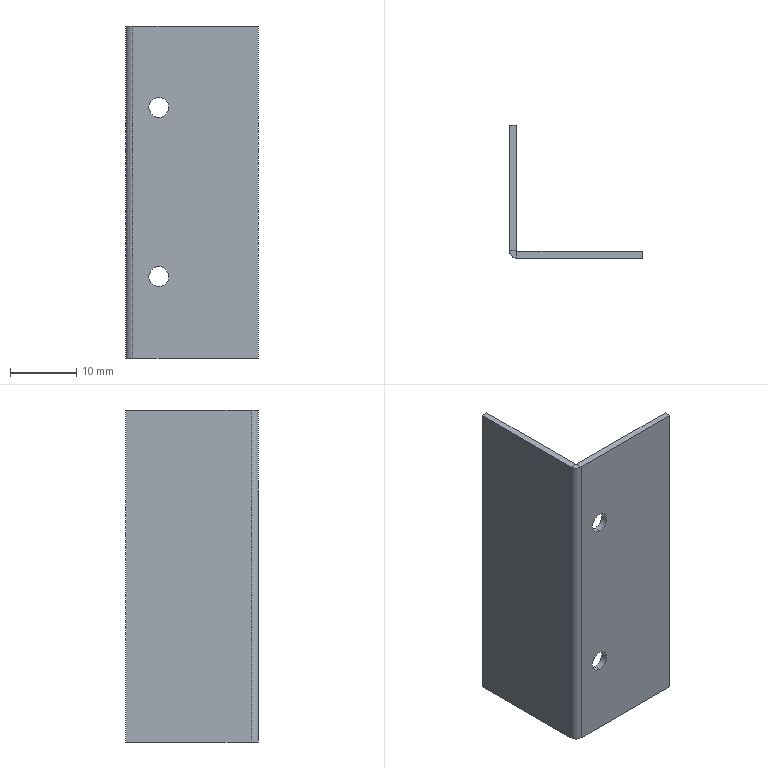Component | SolidWorks | CabinetWelding-1_LimitSwitchBracket-1 | 1 solid | 18 faces | box 20 x 20 x 50 mm | volume 1923 mm3 | plane 12 | cylinder 6 | commonest cylinder face diameters 3 x4 2.2 x1 0.2 x1
STEP:
#1=COLOUR_RGB('',0.7922,0.8196,0.9333);
#2=FILL_AREA_STYLE_COLOUR('',#1);
#3=FILL_AREA_STYLE('',(#2));
#4=SURFACE_STYLE_FILL_AREA(#3);
#5=SURFACE_SIDE_STYLE('',(#4));
#6=SURFACE_STYLE_USAGE(.BOTH.,#5);
#7=PRESENTATION_STYLE_ASSIGNMENT((#6));
#8=CARTESIAN_POINT('',(4.46,33.389,93.238));
#9=VERTEX_POINT('',#8);
#10=CARTESIAN_POINT('',(4.46,33.389,93.357));
#11=VERTEX_POINT('',#10);
#12=CARTESIAN_POINT('',(4.46,33.389,93.297));
#13=DIRECTION('',(-0.,1.,0.));
#14=DIRECTION('',(0.,0.,1.));
#15=AXIS2_PLACEMENT_3D('',#12,#13,#14);
#16=CIRCLE('',#15,0.05906);
#17=EDGE_CURVE('',#9,#11,#16,.T.);
#18=ORIENTED_EDGE('',*,*,#17,.F.);
#19=CARTESIAN_POINT('',(4.46,33.428,93.238));
#20=VERTEX_POINT('',#19);
#21=CARTESIAN_POINT('',(4.46,33.389,93.238));
#22=DIRECTION('',(-0.,1.,0.));
#23=VECTOR('',#22,39.37);
#24=LINE('',#21,#23);
#25=EDGE_CURVE('',#9,#20,#24,.T.);
#26=ORIENTED_EDGE('',*,*,#25,.T.);
#27=CARTESIAN_POINT('',(4.46,33.428,93.357));
#28=VERTEX_POINT('',#27);
#29=CARTESIAN_POINT('',(4.46,33.428,93.297));
#30=DIRECTION('',(-0.,1.,0.));
#31=DIRECTION('',(0.,0.,1.));
#32=AXIS2_PLACEMENT_3D('',#29,#30,#31);
#33=CIRCLE('',#32,0.05906);
#34=EDGE_CURVE('',#20,#28,#33,.T.);
#35=ORIENTED_EDGE('',*,*,#34,.T.);
#36=CARTESIAN_POINT('',(4.46,33.389,93.357));
#37=DIRECTION('',(-0.,1.,0.));
#38=VECTOR('',#37,39.37);
#39=LINE('',#36,#38);
#40=EDGE_CURVE('',#11,#28,#39,.T.);
#41=ORIENTED_EDGE('',*,*,#40,.F.);
#42=EDGE_LOOP('',(#18,#26,#35,#41));
#43=FACE_OUTER_BOUND('',#42,.T.);
#44=CARTESIAN_POINT('',(4.46,33.389,93.297));
#45=DIRECTION('',(-0.,1.,0.));
#46=DIRECTION('',(0.,0.,1.));
#47=AXIS2_PLACEMENT_3D('',#44,#45,#46);
#48=CYLINDRICAL_SURFACE('',#47,0.05906);
#49=ADVANCED_FACE('',(#43),#48,.F.);
#50=CARTESIAN_POINT('',(4.46,33.389,92.234));
#51=VERTEX_POINT('',#50);
#52=CARTESIAN_POINT('',(4.46,33.389,92.353));
#53=VERTEX_POINT('',#52);
#54=CARTESIAN_POINT('',(4.46,33.389,92.294));
#55=DIRECTION('',(-0.,1.,0.));
#56=DIRECTION('',(0.,0.,1.));
#57=AXIS2_PLACEMENT_3D('',#54,#55,#56);
#58=CIRCLE('',#57,0.05906);
#59=EDGE_CURVE('',#51,#53,#58,.T.);
#60=ORIENTED_EDGE('',*,*,#59,.F.);
#61=CARTESIAN_POINT('',(4.46,33.428,92.234));
#62=VERTEX_POINT('',#61);
#63=CARTESIAN_POINT('',(4.46,33.389,92.234));
#64=DIRECTION('',(-0.,1.,0.));
#65=VECTOR('',#64,39.37);
#66=LINE('',#63,#65);
#67=EDGE_CURVE('',#51,#62,#66,.T.);
#68=ORIENTED_EDGE('',*,*,#67,.T.);
#69=CARTESIAN_POINT('',(4.46,33.428,92.353));
#70=VERTEX_POINT('',#69);
#71=CARTESIAN_POINT('',(4.46,33.428,92.294));
#72=DIRECTION('',(-0.,1.,0.));
#73=DIRECTION('',(0.,0.,1.));
#74=AXIS2_PLACEMENT_3D('',#71,#72,#73);
#75=CIRCLE('',#74,0.05906);
#76=EDGE_CURVE('',#62,#70,#75,.T.);
#77=ORIENTED_EDGE('',*,*,#76,.T.);
#78=CARTESIAN_POINT('',(4.46,33.389,92.353));
#79=DIRECTION('',(-0.,1.,0.));
#80=VECTOR('',#79,39.37);
#81=LINE('',#78,#80);
#82=EDGE_CURVE('',#53,#70,#81,.T.);
#83=ORIENTED_EDGE('',*,*,#82,.F.);
#84=EDGE_LOOP('',(#60,#68,#77,#83));
#85=FACE_OUTER_BOUND('',#84,.T.);
#86=CARTESIAN_POINT('',(4.46,33.389,92.294));
#87=DIRECTION('',(-0.,1.,0.));
#88=DIRECTION('',(0.,0.,1.));
#89=AXIS2_PLACEMENT_3D('',#86,#87,#88);
#90=CYLINDRICAL_SURFACE('',#89,0.05906);
#91=ADVANCED_FACE('',(#85),#90,.F.);
#92=CARTESIAN_POINT('',(4.302,33.432,91.811));
#93=VERTEX_POINT('',#92);
#94=CARTESIAN_POINT('',(4.302,34.176,91.811));
#95=VERTEX_POINT('',#94);
#96=CARTESIAN_POINT('',(4.302,34.176,91.811));
#97=DIRECTION('',(-0.,1.,0.));
#98=VECTOR('',#97,39.37);
#99=LINE('',#96,#98);
#100=EDGE_CURVE('',#93,#95,#99,.T.);
#101=ORIENTED_EDGE('',*,*,#100,.F.);
#102=CARTESIAN_POINT('',(4.263,33.432,91.811));
#103=VERTEX_POINT('',#102);
#104=CARTESIAN_POINT('',(4.263,33.432,91.811));
#105=DIRECTION('',(-1.,-0.,0.));
#106=VECTOR('',#105,39.37);
#107=LINE('',#104,#106);
#108=EDGE_CURVE('',#93,#103,#107,.T.);
#109=ORIENTED_EDGE('',*,*,#108,.T.);
#110=CARTESIAN_POINT('',(4.263,34.176,91.811));
#111=VERTEX_POINT('',#110);
#112=CARTESIAN_POINT('',(4.263,34.176,91.811));
#113=DIRECTION('',(-0.,1.,0.));
#114=VECTOR('',#113,39.37);
#115=LINE('',#112,#114);
#116=EDGE_CURVE('',#103,#111,#115,.T.);
#117=ORIENTED_EDGE('',*,*,#116,.T.);
#118=CARTESIAN_POINT('',(4.263,34.176,91.811));
#119=DIRECTION('',(1.,0.,-0.));
#120=VECTOR('',#119,39.37);
#121=LINE('',#118,#120);
#122=EDGE_CURVE('',#111,#95,#121,.T.);
#123=ORIENTED_EDGE('',*,*,#122,.T.);
#124=EDGE_LOOP('',(#101,#109,#117,#123));
#125=FACE_OUTER_BOUND('',#124,.T.);
#126=CARTESIAN_POINT('',(4.263,34.176,91.811));
#127=DIRECTION('',(-0.,0.,-1.));
#128=DIRECTION('',(1.,0.,-0.));
#129=AXIS2_PLACEMENT_3D('',#126,#127,#128);
#130=PLANE('',#129);
#131=ADVANCED_FACE('',(#125),#130,.T.);
#132=CARTESIAN_POINT('',(4.263,34.176,93.78));
#133=VERTEX_POINT('',#132);
#134=CARTESIAN_POINT('',(4.263,33.432,93.78));
#135=VERTEX_POINT('',#134);
#136=CARTESIAN_POINT('',(4.263,32.664,93.78));
#137=DIRECTION('',(0.,-1.,-0.));
#138=VECTOR('',#137,39.37);
#139=LINE('',#136,#138);
#140=EDGE_CURVE('',#133,#135,#139,.T.);
#141=ORIENTED_EDGE('',*,*,#140,.T.);
#142=CARTESIAN_POINT('',(4.302,33.432,93.78));
#143=VERTEX_POINT('',#142);
#144=CARTESIAN_POINT('',(4.263,33.432,93.78));
#145=DIRECTION('',(1.,0.,-0.));
#146=VECTOR('',#145,39.37);
#147=LINE('',#144,#146);
#148=EDGE_CURVE('',#135,#143,#147,.T.);
#149=ORIENTED_EDGE('',*,*,#148,.T.);
#150=CARTESIAN_POINT('',(4.302,34.176,93.78));
#151=VERTEX_POINT('',#150);
#152=CARTESIAN_POINT('',(4.302,32.664,93.78));
#153=DIRECTION('',(0.,-1.,-0.));
#154=VECTOR('',#153,39.37);
#155=LINE('',#152,#154);
#156=EDGE_CURVE('',#151,#143,#155,.T.);
#157=ORIENTED_EDGE('',*,*,#156,.F.);
#158=CARTESIAN_POINT('',(4.263,34.176,93.78));
#159=DIRECTION('',(1.,0.,-0.));
#160=VECTOR('',#159,39.37);
#161=LINE('',#158,#160);
#162=EDGE_CURVE('',#133,#151,#161,.T.);
#163=ORIENTED_EDGE('',*,*,#162,.F.);
#164=EDGE_LOOP('',(#141,#149,#157,#163));
#165=FACE_OUTER_BOUND('',#164,.T.);
#166=CARTESIAN_POINT('',(4.263,32.664,93.78));
#167=DIRECTION('',(0.,-0.,1.));
#168=DIRECTION('',(-1.,-0.,0.));
#169=AXIS2_PLACEMENT_3D('',#166,#167,#168);
#170=PLANE('',#169);
#171=ADVANCED_FACE('',(#165),#170,.T.);
#172=ORIENTED_EDGE('',*,*,#116,.F.);
#173=CARTESIAN_POINT('',(4.263,33.432,-1457.784));
#174=DIRECTION('',(0.,-0.,1.));
#175=VECTOR('',#174,39.37);
#176=LINE('',#173,#175);
#177=EDGE_CURVE('',#103,#135,#176,.T.);
#178=ORIENTED_EDGE('',*,*,#177,.T.);
#179=ORIENTED_EDGE('',*,*,#140,.F.);
#180=CARTESIAN_POINT('',(4.263,34.176,93.78));
#181=DIRECTION('',(0.,-0.,1.));
#182=VECTOR('',#181,39.37);
#183=LINE('',#180,#182);
#184=EDGE_CURVE('',#111,#133,#183,.T.);
#185=ORIENTED_EDGE('',*,*,#184,.F.);
#186=EDGE_LOOP('',(#172,#178,#179,#185));
#187=FACE_OUTER_BOUND('',#186,.T.);
#188=CARTESIAN_POINT('',(4.263,328.409,-1457.784));
#189=DIRECTION('',(-1.,-0.,0.));
#190=DIRECTION('',(-0.,0.,-1.));
#191=AXIS2_PLACEMENT_3D('',#188,#189,#190);
#192=PLANE('',#191);
#193=ADVANCED_FACE('',(#187),#192,.T.);
#194=CARTESIAN_POINT('',(4.302,34.176,93.78));
#195=DIRECTION('',(0.,-0.,1.));
#196=VECTOR('',#195,39.37);
#197=LINE('',#194,#196);
#198=EDGE_CURVE('',#95,#151,#197,.T.);
#199=ORIENTED_EDGE('',*,*,#198,.F.);
#200=ORIENTED_EDGE('',*,*,#122,.F.);
#201=ORIENTED_EDGE('',*,*,#184,.T.);
#202=ORIENTED_EDGE('',*,*,#162,.T.);
#203=EDGE_LOOP('',(#199,#200,#201,#202));
#204=FACE_OUTER_BOUND('',#203,.T.);
#205=CARTESIAN_POINT('',(4.263,34.176,93.78));
#206=DIRECTION('',(-0.,1.,0.));
#207=DIRECTION('',(-1.,-0.,0.));
#208=AXIS2_PLACEMENT_3D('',#205,#206,#207);
#209=PLANE('',#208);
#210=ADVANCED_FACE('',(#204),#209,.T.);
#211=CARTESIAN_POINT('',(4.302,33.432,-1457.784));
#212=DIRECTION('',(0.,-0.,1.));
#213=VECTOR('',#212,39.37);
#214=LINE('',#211,#213);
#215=EDGE_CURVE('',#93,#143,#214,.T.);
#216=ORIENTED_EDGE('',*,*,#215,.F.);
#217=ORIENTED_EDGE('',*,*,#100,.T.);
#218=ORIENTED_EDGE('',*,*,#198,.T.);
#219=ORIENTED_EDGE('',*,*,#156,.T.);
#220=EDGE_LOOP('',(#216,#217,#218,#219));
#221=FACE_OUTER_BOUND('',#220,.T.);
#222=CARTESIAN_POINT('',(4.302,328.409,-1457.784));
#223=DIRECTION('',(-1.,-0.,0.));
#224=DIRECTION('',(-0.,0.,-1.));
#225=AXIS2_PLACEMENT_3D('',#222,#223,#224);
#226=PLANE('',#225);
#227=ADVANCED_FACE('',(#221),#226,.F.);
#228=ORIENTED_EDGE('',*,*,#67,.F.);
#229=CARTESIAN_POINT('',(4.46,33.389,92.294));
#230=DIRECTION('',(-0.,1.,0.));
#231=DIRECTION('',(0.,0.,1.));
#232=AXIS2_PLACEMENT_3D('',#229,#230,#231);
#233=CIRCLE('',#232,0.05906);
#234=EDGE_CURVE('',#53,#51,#233,.T.);
#235=ORIENTED_EDGE('',*,*,#234,.F.);
#236=ORIENTED_EDGE('',*,*,#82,.T.);
#237=CARTESIAN_POINT('',(4.46,33.428,92.294));
#238=DIRECTION('',(-0.,1.,0.));
#239=DIRECTION('',(0.,0.,1.));
#240=AXIS2_PLACEMENT_3D('',#237,#238,#239);
#241=CIRCLE('',#240,0.05906);
#242=EDGE_CURVE('',#70,#62,#241,.T.);
#243=ORIENTED_EDGE('',*,*,#242,.T.);
#244=EDGE_LOOP('',(#228,#235,#236,#243));
#245=FACE_OUTER_BOUND('',#244,.T.);
#246=CARTESIAN_POINT('',(4.46,33.389,92.294));
#247=DIRECTION('',(-0.,1.,0.));
#248=DIRECTION('',(0.,0.,1.));
#249=AXIS2_PLACEMENT_3D('',#246,#247,#248);
#250=CYLINDRICAL_SURFACE('',#249,0.05906);
#251=ADVANCED_FACE('',(#245),#250,.F.);
#252=ORIENTED_EDGE('',*,*,#25,.F.);
#253=CARTESIAN_POINT('',(4.46,33.389,93.297));
#254=DIRECTION('',(-0.,1.,0.));
#255=DIRECTION('',(0.,0.,1.));
#256=AXIS2_PLACEMENT_3D('',#253,#254,#255);
#257=CIRCLE('',#256,0.05906);
#258=EDGE_CURVE('',#11,#9,#257,.T.);
#259=ORIENTED_EDGE('',*,*,#258,.F.);
#260=ORIENTED_EDGE('',*,*,#40,.T.);
#261=CARTESIAN_POINT('',(4.46,33.428,93.297));
#262=DIRECTION('',(-0.,1.,0.));
#263=DIRECTION('',(0.,0.,1.));
#264=AXIS2_PLACEMENT_3D('',#261,#262,#263);
#265=CIRCLE('',#264,0.05906);
#266=EDGE_CURVE('',#28,#20,#265,.T.);
#267=ORIENTED_EDGE('',*,*,#266,.T.);
#268=EDGE_LOOP('',(#252,#259,#260,#267));
#269=FACE_OUTER_BOUND('',#268,.T.);
#270=CARTESIAN_POINT('',(4.46,33.389,93.297));
#271=DIRECTION('',(-0.,1.,0.));
#272=DIRECTION('',(0.,0.,1.));
#273=AXIS2_PLACEMENT_3D('',#270,#271,#272);
#274=CYLINDRICAL_SURFACE('',#273,0.05906);
#275=ADVANCED_FACE('',(#269),#274,.F.);
#276=CARTESIAN_POINT('',(5.05,33.428,93.78));
#277=VERTEX_POINT('',#276);
#278=CARTESIAN_POINT('',(5.05,33.428,91.811));
#279=VERTEX_POINT('',#278);
#280=CARTESIAN_POINT('',(5.05,33.428,91.811));
#281=DIRECTION('',(-0.,0.,-1.));
#282=VECTOR('',#281,39.37);
#283=LINE('',#280,#282);
#284=EDGE_CURVE('',#277,#279,#283,.T.);
#285=ORIENTED_EDGE('',*,*,#284,.F.);
#286=CARTESIAN_POINT('',(5.05,33.389,93.78));
#287=VERTEX_POINT('',#286);
#288=CARTESIAN_POINT('',(5.05,33.389,93.78));
#289=DIRECTION('',(-0.,1.,0.));
#290=VECTOR('',#289,39.37);
#291=LINE('',#288,#290);
#292=EDGE_CURVE('',#287,#277,#291,.T.);
#293=ORIENTED_EDGE('',*,*,#292,.F.);
#294=CARTESIAN_POINT('',(5.05,33.389,91.811));
#295=VERTEX_POINT('',#294);
#296=CARTESIAN_POINT('',(5.05,33.389,91.811));
#297=DIRECTION('',(-0.,0.,-1.));
#298=VECTOR('',#297,39.37);
#299=LINE('',#296,#298);
#300=EDGE_CURVE('',#287,#295,#299,.T.);
#301=ORIENTED_EDGE('',*,*,#300,.T.);
#302=CARTESIAN_POINT('',(5.05,33.389,91.811));
#303=DIRECTION('',(-0.,1.,0.));
#304=VECTOR('',#303,39.37);
#305=LINE('',#302,#304);
#306=EDGE_CURVE('',#295,#279,#305,.T.);
#307=ORIENTED_EDGE('',*,*,#306,.T.);
#308=EDGE_LOOP('',(#285,#293,#301,#307));
#309=FACE_OUTER_BOUND('',#308,.T.);
#310=CARTESIAN_POINT('',(5.05,33.389,91.811));
#311=DIRECTION('',(1.,0.,-0.));
#312=DIRECTION('',(-0.,1.,0.));
#313=AXIS2_PLACEMENT_3D('',#310,#311,#312);
#314=PLANE('',#313);
#315=ADVANCED_FACE('',(#309),#314,.T.);
#316=CARTESIAN_POINT('',(4.306,33.389,91.811));
#317=VERTEX_POINT('',#316);
#318=CARTESIAN_POINT('',(4.306,33.389,93.78));
#319=VERTEX_POINT('',#318);
#320=CARTESIAN_POINT('',(4.306,33.389,-1457.784));
#321=DIRECTION('',(0.,-0.,1.));
#322=VECTOR('',#321,39.37);
#323=LINE('',#320,#322);
#324=EDGE_CURVE('',#317,#319,#323,.T.);
#325=ORIENTED_EDGE('',*,*,#324,.F.);
#326=CARTESIAN_POINT('',(3.539,33.389,91.811));
#327=DIRECTION('',(-1.,-0.,0.));
#328=VECTOR('',#327,39.37);
#329=LINE('',#326,#328);
#330=EDGE_CURVE('',#295,#317,#329,.T.);
#331=ORIENTED_EDGE('',*,*,#330,.F.);
#332=ORIENTED_EDGE('',*,*,#300,.F.);
#333=CARTESIAN_POINT('',(5.05,33.389,93.78));
#334=DIRECTION('',(1.,0.,-0.));
#335=VECTOR('',#334,39.37);
#336=LINE('',#333,#335);
#337=EDGE_CURVE('',#319,#287,#336,.T.);
#338=ORIENTED_EDGE('',*,*,#337,.F.);
#339=EDGE_LOOP('',(#325,#331,#332,#338));
#340=FACE_OUTER_BOUND('',#339,.T.);
#341=ORIENTED_EDGE('',*,*,#258,.T.);
#342=ORIENTED_EDGE('',*,*,#17,.T.);
#343=EDGE_LOOP('',(#341,#342));
#344=FACE_BOUND('',#343,.T.);
#345=ORIENTED_EDGE('',*,*,#234,.T.);
#346=ORIENTED_EDGE('',*,*,#59,.T.);
#347=EDGE_LOOP('',(#345,#346));
#348=FACE_BOUND('',#347,.T.);
#349=CARTESIAN_POINT('',(-290.694,33.389,-1457.784));
#350=DIRECTION('',(0.,-1.,-0.));
#351=DIRECTION('',(-0.,0.,-1.));
#352=AXIS2_PLACEMENT_3D('',#349,#350,#351);
#353=PLANE('',#352);
#354=ADVANCED_FACE('',(#340,#344,#348),#353,.T.);
#355=CARTESIAN_POINT('',(4.306,33.428,91.811));
#356=VERTEX_POINT('',#355);
#357=CARTESIAN_POINT('',(4.306,33.389,91.811));
#358=DIRECTION('',(0.,-1.,-0.));
#359=VECTOR('',#358,39.37);
#360=LINE('',#357,#359);
#361=EDGE_CURVE('',#356,#317,#360,.T.);
#362=ORIENTED_EDGE('',*,*,#361,.F.);
#363=CARTESIAN_POINT('',(3.539,33.428,91.811));
#364=DIRECTION('',(-1.,-0.,0.));
#365=VECTOR('',#364,39.37);
#366=LINE('',#363,#365);
#367=EDGE_CURVE('',#279,#356,#366,.T.);
#368=ORIENTED_EDGE('',*,*,#367,.F.);
#369=ORIENTED_EDGE('',*,*,#306,.F.);
#370=ORIENTED_EDGE('',*,*,#330,.T.);
#371=EDGE_LOOP('',(#362,#368,#369,#370));
#372=FACE_OUTER_BOUND('',#371,.T.);
#373=CARTESIAN_POINT('',(3.539,33.389,91.811));
#374=DIRECTION('',(-0.,0.,-1.));
#375=DIRECTION('',(-0.,1.,0.));
#376=AXIS2_PLACEMENT_3D('',#373,#374,#375);
#377=PLANE('',#376);
#378=ADVANCED_FACE('',(#372),#377,.T.);
#379=ORIENTED_EDGE('',*,*,#242,.F.);
#380=ORIENTED_EDGE('',*,*,#76,.F.);
#381=EDGE_LOOP('',(#379,#380));
#382=FACE_BOUND('',#381,.T.);
#383=ORIENTED_EDGE('',*,*,#266,.F.);
#384=ORIENTED_EDGE('',*,*,#34,.F.);
#385=EDGE_LOOP('',(#383,#384));
#386=FACE_BOUND('',#385,.T.);
#387=ORIENTED_EDGE('',*,*,#367,.T.);
#388=CARTESIAN_POINT('',(4.306,33.428,93.78));
#389=VERTEX_POINT('',#388);
#390=CARTESIAN_POINT('',(4.306,33.428,-1457.784));
#391=DIRECTION('',(0.,-0.,1.));
#392=VECTOR('',#391,39.37);
#393=LINE('',#390,#392);
#394=EDGE_CURVE('',#356,#389,#393,.T.);
#395=ORIENTED_EDGE('',*,*,#394,.T.);
#396=CARTESIAN_POINT('',(5.05,33.428,93.78));
#397=DIRECTION('',(1.,0.,-0.));
#398=VECTOR('',#397,39.37);
#399=LINE('',#396,#398);
#400=EDGE_CURVE('',#389,#277,#399,.T.);
#401=ORIENTED_EDGE('',*,*,#400,.T.);
#402=ORIENTED_EDGE('',*,*,#284,.T.);
#403=EDGE_LOOP('',(#387,#395,#401,#402));
#404=FACE_OUTER_BOUND('',#403,.T.);
#405=CARTESIAN_POINT('',(-290.694,33.428,-1457.784));
#406=DIRECTION('',(0.,-1.,-0.));
#407=DIRECTION('',(-0.,0.,-1.));
#408=AXIS2_PLACEMENT_3D('',#405,#406,#407);
#409=PLANE('',#408);
#410=ADVANCED_FACE('',(#382,#386,#404),#409,.F.);
#411=CARTESIAN_POINT('',(4.306,33.389,93.78));
#412=DIRECTION('',(-0.,1.,0.));
#413=VECTOR('',#412,39.37);
#414=LINE('',#411,#413);
#415=EDGE_CURVE('',#319,#389,#414,.T.);
#416=ORIENTED_EDGE('',*,*,#415,.F.);
#417=ORIENTED_EDGE('',*,*,#337,.T.);
#418=ORIENTED_EDGE('',*,*,#292,.T.);
#419=ORIENTED_EDGE('',*,*,#400,.F.);
#420=EDGE_LOOP('',(#416,#417,#418,#419));
#421=FACE_OUTER_BOUND('',#420,.T.);
#422=CARTESIAN_POINT('',(5.05,33.389,93.78));
#423=DIRECTION('',(0.,-0.,1.));
#424=DIRECTION('',(0.,-1.,-0.));
#425=AXIS2_PLACEMENT_3D('',#422,#423,#424);
#426=PLANE('',#425);
#427=ADVANCED_FACE('',(#421),#426,.T.);
#428=ORIENTED_EDGE('',*,*,#108,.F.);
#429=CARTESIAN_POINT('',(4.306,33.432,91.811));
#430=DIRECTION('',(0.,-0.,1.));
#431=DIRECTION('',(0.,1.,0.));
#432=AXIS2_PLACEMENT_3D('',#429,#430,#431);
#433=CIRCLE('',#432,0.003937);
#434=EDGE_CURVE('',#93,#356,#433,.T.);
#435=ORIENTED_EDGE('',*,*,#434,.T.);
#436=ORIENTED_EDGE('',*,*,#361,.T.);
#437=CARTESIAN_POINT('',(4.306,33.432,91.811));
#438=DIRECTION('',(0.,-0.,1.));
#439=DIRECTION('',(0.,1.,0.));
#440=AXIS2_PLACEMENT_3D('',#437,#438,#439);
#441=CIRCLE('',#440,0.04331);
#442=EDGE_CURVE('',#103,#317,#441,.T.);
#443=ORIENTED_EDGE('',*,*,#442,.F.);
#444=EDGE_LOOP('',(#428,#435,#436,#443));
#445=FACE_OUTER_BOUND('',#444,.T.);
#446=CARTESIAN_POINT('',(4.306,33.432,91.811));
#447=DIRECTION('',(-0.,0.,-1.));
#448=DIRECTION('',(-0.,1.,0.));
#449=AXIS2_PLACEMENT_3D('',#446,#447,#448);
#450=PLANE('',#449);
#451=ADVANCED_FACE('',(#445),#450,.T.);
#452=CARTESIAN_POINT('',(4.306,33.432,93.78));
#453=DIRECTION('',(-0.,0.,-1.));
#454=DIRECTION('',(0.,1.,0.));
#455=AXIS2_PLACEMENT_3D('',#452,#453,#454);
#456=CIRCLE('',#455,0.003937);
#457=EDGE_CURVE('',#389,#143,#456,.T.);
#458=ORIENTED_EDGE('',*,*,#457,.T.);
#459=ORIENTED_EDGE('',*,*,#148,.F.);
#460=CARTESIAN_POINT('',(4.306,33.432,93.78));
#461=DIRECTION('',(-0.,0.,-1.));
#462=DIRECTION('',(0.,-1.,0.));
#463=AXIS2_PLACEMENT_3D('',#460,#461,#462);
#464=CIRCLE('',#463,0.04331);
#465=EDGE_CURVE('',#319,#135,#464,.T.);
#466=ORIENTED_EDGE('',*,*,#465,.F.);
#467=ORIENTED_EDGE('',*,*,#415,.T.);
#468=EDGE_LOOP('',(#458,#459,#466,#467));
#469=FACE_OUTER_BOUND('',#468,.T.);
#470=CARTESIAN_POINT('',(4.306,33.432,93.78));
#471=DIRECTION('',(0.,-0.,1.));
#472=DIRECTION('',(0.,-1.,-0.));
#473=AXIS2_PLACEMENT_3D('',#470,#471,#472);
#474=PLANE('',#473);
#475=ADVANCED_FACE('',(#469),#474,.T.);
#476=ORIENTED_EDGE('',*,*,#324,.T.);
#477=ORIENTED_EDGE('',*,*,#465,.T.);
#478=ORIENTED_EDGE('',*,*,#177,.F.);
#479=ORIENTED_EDGE('',*,*,#442,.T.);
#480=EDGE_LOOP('',(#476,#477,#478,#479));
#481=FACE_OUTER_BOUND('',#480,.T.);
#482=CARTESIAN_POINT('',(4.306,33.432,94.765));
#483=DIRECTION('',(-0.,0.,-1.));
#484=DIRECTION('',(0.,1.,0.));
#485=AXIS2_PLACEMENT_3D('',#482,#483,#484);
#486=CYLINDRICAL_SURFACE('',#485,0.04331);
#487=ADVANCED_FACE('',(#481),#486,.T.);
#488=ORIENTED_EDGE('',*,*,#394,.F.);
#489=ORIENTED_EDGE('',*,*,#434,.F.);
#490=ORIENTED_EDGE('',*,*,#215,.T.);
#491=ORIENTED_EDGE('',*,*,#457,.F.);
#492=EDGE_LOOP('',(#488,#489,#490,#491));
#493=FACE_OUTER_BOUND('',#492,.T.);
#494=CARTESIAN_POINT('',(4.306,33.432,94.765));
#495=DIRECTION('',(-0.,0.,-1.));
#496=DIRECTION('',(0.,1.,0.));
#497=AXIS2_PLACEMENT_3D('',#494,#495,#496);
#498=CYLINDRICAL_SURFACE('',#497,0.003937);
#499=ADVANCED_FACE('',(#493),#498,.F.);
#500=CLOSED_SHELL('',(#49,#91,#131,#171,#193,#210,#227,#251,#275,#315,#354,#378,#410,#427,#451,#475,#487,#499));
#501=MANIFOLD_SOLID_BREP('',#500);
#502=STYLED_ITEM('',(#7),#501);
#503=PRESENTATION_LAYER_ASSIGNMENT('','',(#502));
#504=(LENGTH_UNIT()NAMED_UNIT(*)SI_UNIT($,.METRE.));
#505=LENGTH_MEASURE_WITH_UNIT(LENGTH_MEASURE(0.0254),#504);
#506=DIMENSIONAL_EXPONENTS(1.,0.,0.,0.,0.,0.,0.);
#507=(CONVERSION_BASED_UNIT('',#505)LENGTH_UNIT()NAMED_UNIT(#506));
#508=UNCERTAINTY_MEASURE_WITH_UNIT(LENGTH_MEASURE(0.00001),#507,'','');
#509=(NAMED_UNIT(*)PLANE_ANGLE_UNIT()SI_UNIT($,.RADIAN.));
#510=(NAMED_UNIT(*)SI_UNIT($,.STERADIAN.)SOLID_ANGLE_UNIT());
#511=(GEOMETRIC_REPRESENTATION_CONTEXT(3)GLOBAL_UNCERTAINTY_ASSIGNED_CONTEXT((#508))GLOBAL_UNIT_ASSIGNED_CONTEXT((#507,#509,#510))REPRESENTATION_CONTEXT('',''));
#512=MECHANICAL_DESIGN_GEOMETRIC_PRESENTATION_REPRESENTATION('',(#502),#511);
#513=CARTESIAN_POINT('',(0.,0.,0.));
#514=DIRECTION('',(0.,0.,1.));
#515=DIRECTION('',(1.,0.,0.));
#516=AXIS2_PLACEMENT_3D('',#513,#514,#515);
#517=(LENGTH_UNIT()NAMED_UNIT(*)SI_UNIT($,.METRE.));
#518=LENGTH_MEASURE_WITH_UNIT(LENGTH_MEASURE(0.0254),#517);
#519=DIMENSIONAL_EXPONENTS(1.,0.,0.,0.,0.,0.,0.);
#520=(CONVERSION_BASED_UNIT('',#518)LENGTH_UNIT()NAMED_UNIT(#519));
#521=UNCERTAINTY_MEASURE_WITH_UNIT(LENGTH_MEASURE(0.00001),#520,'','');
#522=(NAMED_UNIT(*)PLANE_ANGLE_UNIT()SI_UNIT($,.RADIAN.));
#523=(NAMED_UNIT(*)SI_UNIT($,.STERADIAN.)SOLID_ANGLE_UNIT());
#524=(GEOMETRIC_REPRESENTATION_CONTEXT(3)GLOBAL_UNCERTAINTY_ASSIGNED_CONTEXT((#521))GLOBAL_UNIT_ASSIGNED_CONTEXT((#520,#522,#523))REPRESENTATION_CONTEXT('',''));
#525=ADVANCED_BREP_SHAPE_REPRESENTATION('',(#501,#516),#524);